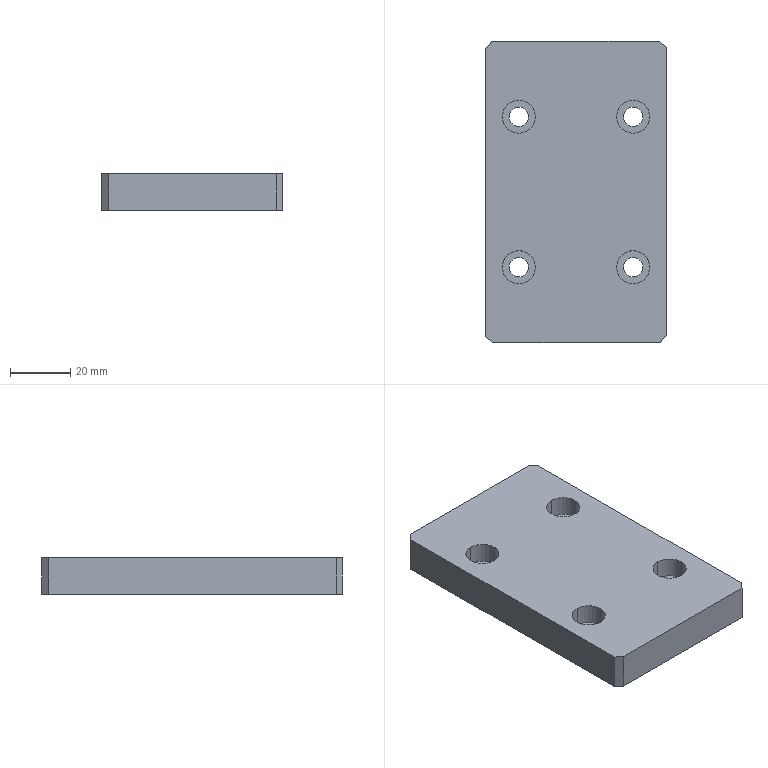Component | SolidWorks | RobotArmSupportPlate-1 | 1 solid | 30 faces | box 60 x 100 x 12 mm | volume 68632 mm3 | cylinder 16 | plane 14 | commonest cylinder face diameters 11 x8 6.4 x8
build123d program:
from build123d import *
from OCP.BRepFilletAPI import BRepFilletAPI_MakeChamfer

# Parameters (mm, degrees)
SKETCH1_W                                           = 100
SKETCH1_H                                           = 60
BOSS_EXTRUDE1_DEPTH                                 = 12
CHAMFER1_SIZE                                       = 2
CHAMFER1_SIZE2                                      = 2.384
HOLE_SIZE_ACCORDING_TO_TYPE2_OF_HEXAGON_D           = 6.4
HOLE_SIZE_ACCORDING_TO_TYPE2_OF_HEXAGON_DEPTH       = 15
HOLE_SIZE_ACCORDING_TO_TYPE2_OF_HEXAGON_CBORE_D     = 11
HOLE_SIZE_ACCORDING_TO_TYPE2_OF_HEXAGON_CBORE_DEPTH = 6.8
HOLE_SIZE_ACCORDING_TO_TYPE2_OF_HEXAGON_TIP         = 1.923


with BuildPart() as part:
    # Sketch1 → Boss-Extrude1 (new body)
    with BuildSketch(Plane.XY):
        Rectangle(SKETCH1_W, SKETCH1_H)
    extrude(amount=BOSS_EXTRUDE1_DEPTH)

    # Chamfer1: one chamfer whose edges measure the first distance from different faces: ONE call of the kernel's chamfer builder (chamfer() names one face for all edges)
    chamfer1_edges_1 = [part.edges().sort_by_distance(p)[0] for p in [
        (50, -30, 6),
    ]]
    chamfer1_side_1 = [part.faces().sort_by_distance(p)[0] for p in [
        (0, -30, 6),
    ]]
    chamfer1_edges_2 = [part.edges().sort_by_distance(p)[0] for p in [
        (-50, -30, 6),
    ]]
    chamfer1_side_2 = [part.faces().sort_by_distance(p)[0] for p in [
        (-50, 0, 6),
    ]]
    chamfer1_edges_3 = [part.edges().sort_by_distance(p)[0] for p in [
        (-50, 30, 6),
    ]]
    chamfer1_side_3 = [part.faces().sort_by_distance(p)[0] for p in [
        (0, 30, 6),
    ]]
    chamfer1_edges_4 = [part.edges().sort_by_distance(p)[0] for p in [
        (50, 30, 6),
    ]]
    chamfer1_side_4 = [part.faces().sort_by_distance(p)[0] for p in [
        (50, 0, 6),
    ]]
    chamfer1 = BRepFilletAPI_MakeChamfer(part.part.solid().wrapped)
    for e in chamfer1_edges_1:
        chamfer1.Add(CHAMFER1_SIZE, CHAMFER1_SIZE2, e.wrapped, chamfer1_side_1[0].wrapped)  # the first distance lies on this face
    for e in chamfer1_edges_2:
        chamfer1.Add(CHAMFER1_SIZE, CHAMFER1_SIZE2, e.wrapped, chamfer1_side_2[0].wrapped)  # the first distance lies on this face
    for e in chamfer1_edges_3:
        chamfer1.Add(CHAMFER1_SIZE, CHAMFER1_SIZE2, e.wrapped, chamfer1_side_3[0].wrapped)  # the first distance lies on this face
    for e in chamfer1_edges_4:
        chamfer1.Add(CHAMFER1_SIZE, CHAMFER1_SIZE2, e.wrapped, chamfer1_side_4[0].wrapped)  # the first distance lies on this face
    add(Compound.cast(chamfer1.Shape()), mode=Mode.REPLACE)

    # Hole Size_According to_Type2 of Hexagon
    with Locations(Plane.XY.offset(12)):
        with Locations((-25, 19), (-25, -19), (25, 19), (25, -19)):
            CounterBoreHole(HOLE_SIZE_ACCORDING_TO_TYPE2_OF_HEXAGON_D / 2, HOLE_SIZE_ACCORDING_TO_TYPE2_OF_HEXAGON_CBORE_D / 2, HOLE_SIZE_ACCORDING_TO_TYPE2_OF_HEXAGON_CBORE_DEPTH, depth=HOLE_SIZE_ACCORDING_TO_TYPE2_OF_HEXAGON_DEPTH)
            with Locations((0, 0, -(HOLE_SIZE_ACCORDING_TO_TYPE2_OF_HEXAGON_DEPTH + HOLE_SIZE_ACCORDING_TO_TYPE2_OF_HEXAGON_TIP / 2))):  # 118° drill point
                Cone(0, HOLE_SIZE_ACCORDING_TO_TYPE2_OF_HEXAGON_D / 2, HOLE_SIZE_ACCORDING_TO_TYPE2_OF_HEXAGON_TIP, mode=Mode.SUBTRACT)


solid = part.part

# Placed as in the assembly
solid = solid.moved(Location((-45.522, 19.945, 48.551), (0, 0, 90)))
STEP:
#1=COLOUR_RGB('',0.7922,0.8196,0.9333);
#2=FILL_AREA_STYLE_COLOUR('',#1);
#3=FILL_AREA_STYLE('',(#2));
#4=SURFACE_STYLE_FILL_AREA(#3);
#5=SURFACE_SIDE_STYLE('',(#4));
#6=SURFACE_STYLE_USAGE(.BOTH.,#5);
#7=PRESENTATION_STYLE_ASSIGNMENT((#6));
#8=CARTESIAN_POINT('',(-1.044,1.986,2.116));
#9=VERTEX_POINT('',#8);
#10=CARTESIAN_POINT('',(-1.044,1.553,2.116));
#11=VERTEX_POINT('',#10);
#12=CARTESIAN_POINT('',(-1.044,1.77,2.116));
#13=DIRECTION('',(0.,-0.,1.));
#14=DIRECTION('',(0.,-1.,0.));
#15=AXIS2_PLACEMENT_3D('',#12,#13,#14);
#16=CIRCLE('',#15,0.2165);
#17=EDGE_CURVE('',#9,#11,#16,.T.);
#18=ORIENTED_EDGE('',*,*,#17,.F.);
#19=CARTESIAN_POINT('',(-1.044,1.986,2.384));
#20=VERTEX_POINT('',#19);
#21=CARTESIAN_POINT('',(-1.044,1.986,2.384));
#22=DIRECTION('',(0.,-0.,1.));
#23=VECTOR('',#22,39.37);
#24=LINE('',#21,#23);
#25=EDGE_CURVE('',#9,#20,#24,.T.);
#26=ORIENTED_EDGE('',*,*,#25,.T.);
#27=CARTESIAN_POINT('',(-1.044,1.553,2.384));
#28=VERTEX_POINT('',#27);
#29=CARTESIAN_POINT('',(-1.044,1.77,2.384));
#30=DIRECTION('',(0.,-0.,1.));
#31=DIRECTION('',(0.,-1.,0.));
#32=AXIS2_PLACEMENT_3D('',#29,#30,#31);
#33=CIRCLE('',#32,0.2165);
#34=EDGE_CURVE('',#20,#28,#33,.T.);
#35=ORIENTED_EDGE('',*,*,#34,.T.);
#36=CARTESIAN_POINT('',(-1.044,1.553,2.384));
#37=DIRECTION('',(0.,-0.,1.));
#38=VECTOR('',#37,39.37);
#39=LINE('',#36,#38);
#40=EDGE_CURVE('',#11,#28,#39,.T.);
#41=ORIENTED_EDGE('',*,*,#40,.F.);
#42=EDGE_LOOP('',(#18,#26,#35,#41));
#43=FACE_OUTER_BOUND('',#42,.T.);
#44=CARTESIAN_POINT('',(-1.044,1.77,2.384));
#45=DIRECTION('',(0.,-0.,1.));
#46=DIRECTION('',(0.,-1.,0.));
#47=AXIS2_PLACEMENT_3D('',#44,#45,#46);
#48=CYLINDRICAL_SURFACE('',#47,0.2165);
#49=ADVANCED_FACE('',(#43),#48,.F.);
#50=CARTESIAN_POINT('',(-1.044,1.895,1.911));
#51=VERTEX_POINT('',#50);
#52=CARTESIAN_POINT('',(-1.044,1.644,1.911));
#53=VERTEX_POINT('',#52);
#54=CARTESIAN_POINT('',(-1.044,1.77,1.911));
#55=DIRECTION('',(0.,-0.,1.));
#56=DIRECTION('',(0.,-1.,0.));
#57=AXIS2_PLACEMENT_3D('',#54,#55,#56);
#58=CIRCLE('',#57,0.126);
#59=EDGE_CURVE('',#51,#53,#58,.T.);
#60=ORIENTED_EDGE('',*,*,#59,.F.);
#61=CARTESIAN_POINT('',(-1.044,1.895,2.116));
#62=VERTEX_POINT('',#61);
#63=CARTESIAN_POINT('',(-1.044,1.895,2.384));
#64=DIRECTION('',(0.,-0.,1.));
#65=VECTOR('',#64,39.37);
#66=LINE('',#63,#65);
#67=EDGE_CURVE('',#51,#62,#66,.T.);
#68=ORIENTED_EDGE('',*,*,#67,.T.);
#69=CARTESIAN_POINT('',(-1.044,1.644,2.116));
#70=VERTEX_POINT('',#69);
#71=CARTESIAN_POINT('',(-1.044,1.77,2.116));
#72=DIRECTION('',(0.,-0.,1.));
#73=DIRECTION('',(0.,-1.,0.));
#74=AXIS2_PLACEMENT_3D('',#71,#72,#73);
#75=CIRCLE('',#74,0.126);
#76=EDGE_CURVE('',#62,#70,#75,.T.);
#77=ORIENTED_EDGE('',*,*,#76,.T.);
#78=CARTESIAN_POINT('',(-1.044,1.644,2.384));
#79=DIRECTION('',(0.,-0.,1.));
#80=VECTOR('',#79,39.37);
#81=LINE('',#78,#80);
#82=EDGE_CURVE('',#53,#70,#81,.T.);
#83=ORIENTED_EDGE('',*,*,#82,.F.);
#84=EDGE_LOOP('',(#60,#68,#77,#83));
#85=FACE_OUTER_BOUND('',#84,.T.);
#86=CARTESIAN_POINT('',(-1.044,1.77,2.384));
#87=DIRECTION('',(0.,-0.,1.));
#88=DIRECTION('',(0.,-1.,0.));
#89=AXIS2_PLACEMENT_3D('',#86,#87,#88);
#90=CYLINDRICAL_SURFACE('',#89,0.126);
#91=ADVANCED_FACE('',(#85),#90,.F.);
#92=CARTESIAN_POINT('',(-2.54,1.986,2.116));
#93=VERTEX_POINT('',#92);
#94=CARTESIAN_POINT('',(-2.54,1.553,2.116));
#95=VERTEX_POINT('',#94);
#96=CARTESIAN_POINT('',(-2.54,1.77,2.116));
#97=DIRECTION('',(0.,-0.,1.));
#98=DIRECTION('',(0.,-1.,0.));
#99=AXIS2_PLACEMENT_3D('',#96,#97,#98);
#100=CIRCLE('',#99,0.2165);
#101=EDGE_CURVE('',#93,#95,#100,.T.);
#102=ORIENTED_EDGE('',*,*,#101,.F.);
#103=CARTESIAN_POINT('',(-2.54,1.986,2.384));
#104=VERTEX_POINT('',#103);
#105=CARTESIAN_POINT('',(-2.54,1.986,2.384));
#106=DIRECTION('',(0.,-0.,1.));
#107=VECTOR('',#106,39.37);
#108=LINE('',#105,#107);
#109=EDGE_CURVE('',#93,#104,#108,.T.);
#110=ORIENTED_EDGE('',*,*,#109,.T.);
#111=CARTESIAN_POINT('',(-2.54,1.553,2.384));
#112=VERTEX_POINT('',#111);
#113=CARTESIAN_POINT('',(-2.54,1.77,2.384));
#114=DIRECTION('',(0.,-0.,1.));
#115=DIRECTION('',(0.,-1.,0.));
#116=AXIS2_PLACEMENT_3D('',#113,#114,#115);
#117=CIRCLE('',#116,0.2165);
#118=EDGE_CURVE('',#104,#112,#117,.T.);
#119=ORIENTED_EDGE('',*,*,#118,.T.);
#120=CARTESIAN_POINT('',(-2.54,1.553,2.384));
#121=DIRECTION('',(0.,-0.,1.));
#122=VECTOR('',#121,39.37);
#123=LINE('',#120,#122);
#124=EDGE_CURVE('',#95,#112,#123,.T.);
#125=ORIENTED_EDGE('',*,*,#124,.F.);
#126=EDGE_LOOP('',(#102,#110,#119,#125));
#127=FACE_OUTER_BOUND('',#126,.T.);
#128=CARTESIAN_POINT('',(-2.54,1.77,2.384));
#129=DIRECTION('',(0.,-0.,1.));
#130=DIRECTION('',(0.,-1.,0.));
#131=AXIS2_PLACEMENT_3D('',#128,#129,#130);
#132=CYLINDRICAL_SURFACE('',#131,0.2165);
#133=ADVANCED_FACE('',(#127),#132,.F.);
#134=CARTESIAN_POINT('',(-2.54,1.895,1.911));
#135=VERTEX_POINT('',#134);
#136=CARTESIAN_POINT('',(-2.54,1.644,1.911));
#137=VERTEX_POINT('',#136);
#138=CARTESIAN_POINT('',(-2.54,1.77,1.911));
#139=DIRECTION('',(0.,-0.,1.));
#140=DIRECTION('',(0.,-1.,0.));
#141=AXIS2_PLACEMENT_3D('',#138,#139,#140);
#142=CIRCLE('',#141,0.126);
#143=EDGE_CURVE('',#135,#137,#142,.T.);
#144=ORIENTED_EDGE('',*,*,#143,.F.);
#145=CARTESIAN_POINT('',(-2.54,1.895,2.116));
#146=VERTEX_POINT('',#145);
#147=CARTESIAN_POINT('',(-2.54,1.895,2.384));
#148=DIRECTION('',(0.,-0.,1.));
#149=VECTOR('',#148,39.37);
#150=LINE('',#147,#149);
#151=EDGE_CURVE('',#135,#146,#150,.T.);
#152=ORIENTED_EDGE('',*,*,#151,.T.);
#153=CARTESIAN_POINT('',(-2.54,1.644,2.116));
#154=VERTEX_POINT('',#153);
#155=CARTESIAN_POINT('',(-2.54,1.77,2.116));
#156=DIRECTION('',(0.,-0.,1.));
#157=DIRECTION('',(0.,-1.,0.));
#158=AXIS2_PLACEMENT_3D('',#155,#156,#157);
#159=CIRCLE('',#158,0.126);
#160=EDGE_CURVE('',#146,#154,#159,.T.);
#161=ORIENTED_EDGE('',*,*,#160,.T.);
#162=CARTESIAN_POINT('',(-2.54,1.644,2.384));
#163=DIRECTION('',(0.,-0.,1.));
#164=VECTOR('',#163,39.37);
#165=LINE('',#162,#164);
#166=EDGE_CURVE('',#137,#154,#165,.T.);
#167=ORIENTED_EDGE('',*,*,#166,.F.);
#168=EDGE_LOOP('',(#144,#152,#161,#167));
#169=FACE_OUTER_BOUND('',#168,.T.);
#170=CARTESIAN_POINT('',(-2.54,1.77,2.384));
#171=DIRECTION('',(0.,-0.,1.));
#172=DIRECTION('',(0.,-1.,0.));
#173=AXIS2_PLACEMENT_3D('',#170,#171,#172);
#174=CYLINDRICAL_SURFACE('',#173,0.126);
#175=ADVANCED_FACE('',(#169),#174,.F.);
#176=CARTESIAN_POINT('',(-1.044,0.01754,2.116));
#177=VERTEX_POINT('',#176);
#178=CARTESIAN_POINT('',(-1.044,-0.4155,2.116));
#179=VERTEX_POINT('',#178);
#180=CARTESIAN_POINT('',(-1.044,-0.199,2.116));
#181=DIRECTION('',(0.,-0.,1.));
#182=DIRECTION('',(0.,-1.,0.));
#183=AXIS2_PLACEMENT_3D('',#180,#181,#182);
#184=CIRCLE('',#183,0.2165);
#185=EDGE_CURVE('',#177,#179,#184,.T.);
#186=ORIENTED_EDGE('',*,*,#185,.F.);
#187=CARTESIAN_POINT('',(-1.044,0.01754,2.384));
#188=VERTEX_POINT('',#187);
#189=CARTESIAN_POINT('',(-1.044,0.01754,2.384));
#190=DIRECTION('',(0.,-0.,1.));
#191=VECTOR('',#190,39.37);
#192=LINE('',#189,#191);
#193=EDGE_CURVE('',#177,#188,#192,.T.);
#194=ORIENTED_EDGE('',*,*,#193,.T.);
#195=CARTESIAN_POINT('',(-1.044,-0.4155,2.384));
#196=VERTEX_POINT('',#195);
#197=CARTESIAN_POINT('',(-1.044,-0.199,2.384));
#198=DIRECTION('',(0.,-0.,1.));
#199=DIRECTION('',(0.,-1.,0.));
#200=AXIS2_PLACEMENT_3D('',#197,#198,#199);
#201=CIRCLE('',#200,0.2165);
#202=EDGE_CURVE('',#188,#196,#201,.T.);
#203=ORIENTED_EDGE('',*,*,#202,.T.);
#204=CARTESIAN_POINT('',(-1.044,-0.4155,2.384));
#205=DIRECTION('',(0.,-0.,1.));
#206=VECTOR('',#205,39.37);
#207=LINE('',#204,#206);
#208=EDGE_CURVE('',#179,#196,#207,.T.);
#209=ORIENTED_EDGE('',*,*,#208,.F.);
#210=EDGE_LOOP('',(#186,#194,#203,#209));
#211=FACE_OUTER_BOUND('',#210,.T.);
#212=CARTESIAN_POINT('',(-1.044,-0.199,2.384));
#213=DIRECTION('',(0.,-0.,1.));
#214=DIRECTION('',(0.,-1.,0.));
#215=AXIS2_PLACEMENT_3D('',#212,#213,#214);
#216=CYLINDRICAL_SURFACE('',#215,0.2165);
#217=ADVANCED_FACE('',(#211),#216,.F.);
#218=CARTESIAN_POINT('',(-1.044,-0.07302,1.911));
#219=VERTEX_POINT('',#218);
#220=CARTESIAN_POINT('',(-1.044,-0.325,1.911));
#221=VERTEX_POINT('',#220);
#222=CARTESIAN_POINT('',(-1.044,-0.199,1.911));
#223=DIRECTION('',(0.,-0.,1.));
#224=DIRECTION('',(0.,-1.,0.));
#225=AXIS2_PLACEMENT_3D('',#222,#223,#224);
#226=CIRCLE('',#225,0.126);
#227=EDGE_CURVE('',#219,#221,#226,.T.);
#228=ORIENTED_EDGE('',*,*,#227,.F.);
#229=CARTESIAN_POINT('',(-1.044,-0.07302,2.116));
#230=VERTEX_POINT('',#229);
#231=CARTESIAN_POINT('',(-1.044,-0.07302,2.384));
#232=DIRECTION('',(0.,-0.,1.));
#233=VECTOR('',#232,39.37);
#234=LINE('',#231,#233);
#235=EDGE_CURVE('',#219,#230,#234,.T.);
#236=ORIENTED_EDGE('',*,*,#235,.T.);
#237=CARTESIAN_POINT('',(-1.044,-0.325,2.116));
#238=VERTEX_POINT('',#237);
#239=CARTESIAN_POINT('',(-1.044,-0.199,2.116));
#240=DIRECTION('',(0.,-0.,1.));
#241=DIRECTION('',(0.,-1.,0.));
#242=AXIS2_PLACEMENT_3D('',#239,#240,#241);
#243=CIRCLE('',#242,0.126);
#244=EDGE_CURVE('',#230,#238,#243,.T.);
#245=ORIENTED_EDGE('',*,*,#244,.T.);
#246=CARTESIAN_POINT('',(-1.044,-0.325,2.384));
#247=DIRECTION('',(0.,-0.,1.));
#248=VECTOR('',#247,39.37);
#249=LINE('',#246,#248);
#250=EDGE_CURVE('',#221,#238,#249,.T.);
#251=ORIENTED_EDGE('',*,*,#250,.F.);
#252=EDGE_LOOP('',(#228,#236,#245,#251));
#253=FACE_OUTER_BOUND('',#252,.T.);
#254=CARTESIAN_POINT('',(-1.044,-0.199,2.384));
#255=DIRECTION('',(0.,-0.,1.));
#256=DIRECTION('',(0.,-1.,0.));
#257=AXIS2_PLACEMENT_3D('',#254,#255,#256);
#258=CYLINDRICAL_SURFACE('',#257,0.126);
#259=ADVANCED_FACE('',(#253),#258,.F.);
#260=CARTESIAN_POINT('',(-2.54,0.01754,2.116));
#261=VERTEX_POINT('',#260);
#262=CARTESIAN_POINT('',(-2.54,-0.4155,2.116));
#263=VERTEX_POINT('',#262);
#264=CARTESIAN_POINT('',(-2.54,-0.199,2.116));
#265=DIRECTION('',(0.,-0.,1.));
#266=DIRECTION('',(0.,-1.,0.));
#267=AXIS2_PLACEMENT_3D('',#264,#265,#266);
#268=CIRCLE('',#267,0.2165);
#269=EDGE_CURVE('',#261,#263,#268,.T.);
#270=ORIENTED_EDGE('',*,*,#269,.F.);
#271=CARTESIAN_POINT('',(-2.54,0.01754,2.384));
#272=VERTEX_POINT('',#271);
#273=CARTESIAN_POINT('',(-2.54,0.01754,2.384));
#274=DIRECTION('',(0.,-0.,1.));
#275=VECTOR('',#274,39.37);
#276=LINE('',#273,#275);
#277=EDGE_CURVE('',#261,#272,#276,.T.);
#278=ORIENTED_EDGE('',*,*,#277,.T.);
#279=CARTESIAN_POINT('',(-2.54,-0.4155,2.384));
#280=VERTEX_POINT('',#279);
#281=CARTESIAN_POINT('',(-2.54,-0.199,2.384));
#282=DIRECTION('',(0.,-0.,1.));
#283=DIRECTION('',(0.,-1.,0.));
#284=AXIS2_PLACEMENT_3D('',#281,#282,#283);
#285=CIRCLE('',#284,0.2165);
#286=EDGE_CURVE('',#272,#280,#285,.T.);
#287=ORIENTED_EDGE('',*,*,#286,.T.);
#288=CARTESIAN_POINT('',(-2.54,-0.4155,2.384));
#289=DIRECTION('',(0.,-0.,1.));
#290=VECTOR('',#289,39.37);
#291=LINE('',#288,#290);
#292=EDGE_CURVE('',#263,#280,#291,.T.);
#293=ORIENTED_EDGE('',*,*,#292,.F.);
#294=EDGE_LOOP('',(#270,#278,#287,#293));
#295=FACE_OUTER_BOUND('',#294,.T.);
#296=CARTESIAN_POINT('',(-2.54,-0.199,2.384));
#297=DIRECTION('',(0.,-0.,1.));
#298=DIRECTION('',(0.,-1.,0.));
#299=AXIS2_PLACEMENT_3D('',#296,#297,#298);
#300=CYLINDRICAL_SURFACE('',#299,0.2165);
#301=ADVANCED_FACE('',(#295),#300,.F.);
#302=CARTESIAN_POINT('',(-2.54,-0.07302,1.911));
#303=VERTEX_POINT('',#302);
#304=CARTESIAN_POINT('',(-2.54,-0.325,1.911));
#305=VERTEX_POINT('',#304);
#306=CARTESIAN_POINT('',(-2.54,-0.199,1.911));
#307=DIRECTION('',(0.,-0.,1.));
#308=DIRECTION('',(0.,-1.,0.));
#309=AXIS2_PLACEMENT_3D('',#306,#307,#308);
#310=CIRCLE('',#309,0.126);
#311=EDGE_CURVE('',#303,#305,#310,.T.);
#312=ORIENTED_EDGE('',*,*,#311,.F.);
#313=CARTESIAN_POINT('',(-2.54,-0.07302,2.116));
#314=VERTEX_POINT('',#313);
#315=CARTESIAN_POINT('',(-2.54,-0.07302,2.384));
#316=DIRECTION('',(0.,-0.,1.));
#317=VECTOR('',#316,39.37);
#318=LINE('',#315,#317);
#319=EDGE_CURVE('',#303,#314,#318,.T.);
#320=ORIENTED_EDGE('',*,*,#319,.T.);
#321=CARTESIAN_POINT('',(-2.54,-0.325,2.116));
#322=VERTEX_POINT('',#321);
#323=CARTESIAN_POINT('',(-2.54,-0.199,2.116));
#324=DIRECTION('',(0.,-0.,1.));
#325=DIRECTION('',(0.,-1.,0.));
#326=AXIS2_PLACEMENT_3D('',#323,#324,#325);
#327=CIRCLE('',#326,0.126);
#328=EDGE_CURVE('',#314,#322,#327,.T.);
#329=ORIENTED_EDGE('',*,*,#328,.T.);
#330=CARTESIAN_POINT('',(-2.54,-0.325,2.384));
#331=DIRECTION('',(0.,-0.,1.));
#332=VECTOR('',#331,39.37);
#333=LINE('',#330,#332);
#334=EDGE_CURVE('',#305,#322,#333,.T.);
#335=ORIENTED_EDGE('',*,*,#334,.F.);
#336=EDGE_LOOP('',(#312,#320,#329,#335));
#337=FACE_OUTER_BOUND('',#336,.T.);
#338=CARTESIAN_POINT('',(-2.54,-0.199,2.384));
#339=DIRECTION('',(0.,-0.,1.));
#340=DIRECTION('',(0.,-1.,0.));
#341=AXIS2_PLACEMENT_3D('',#338,#339,#340);
#342=CYLINDRICAL_SURFACE('',#341,0.126);
#343=ADVANCED_FACE('',(#337),#342,.F.);
#344=CARTESIAN_POINT('',(-2.879,-1.183,2.384));
#345=VERTEX_POINT('',#344);
#346=CARTESIAN_POINT('',(-0.6899,-1.183,2.384));
#347=VERTEX_POINT('',#346);
#348=CARTESIAN_POINT('',(-0.6111,-1.183,2.384));
#349=DIRECTION('',(1.,0.,-0.));
#350=VECTOR('',#349,39.37);
#351=LINE('',#348,#350);
#352=EDGE_CURVE('',#345,#347,#351,.T.);
#353=ORIENTED_EDGE('',*,*,#352,.F.);
#354=CARTESIAN_POINT('',(-2.879,-1.183,1.911));
#355=VERTEX_POINT('',#354);
#356=CARTESIAN_POINT('',(-2.879,-1.183,2.384));
#357=DIRECTION('',(-0.,0.,-1.));
#358=VECTOR('',#357,39.37);
#359=LINE('',#356,#358);
#360=EDGE_CURVE('',#345,#355,#359,.T.);
#361=ORIENTED_EDGE('',*,*,#360,.T.);
#362=CARTESIAN_POINT('',(-0.6899,-1.183,1.911));
#363=VERTEX_POINT('',#362);
#364=CARTESIAN_POINT('',(-0.6111,-1.183,1.911));
#365=DIRECTION('',(1.,0.,-0.));
#366=VECTOR('',#365,39.37);
#367=LINE('',#364,#366);
#368=EDGE_CURVE('',#355,#363,#367,.T.);
#369=ORIENTED_EDGE('',*,*,#368,.T.);
#370=CARTESIAN_POINT('',(-0.6899,-1.183,2.384));
#371=DIRECTION('',(0.,-0.,1.));
#372=VECTOR('',#371,39.37);
#373=LINE('',#370,#372);
#374=EDGE_CURVE('',#363,#347,#373,.T.);
#375=ORIENTED_EDGE('',*,*,#374,.T.);
#376=EDGE_LOOP('',(#353,#361,#369,#375));
#377=FACE_OUTER_BOUND('',#376,.T.);
#378=CARTESIAN_POINT('',(-0.6111,-1.183,2.384));
#379=DIRECTION('',(-0.,1.,0.));
#380=DIRECTION('',(-1.,-0.,0.));
#381=AXIS2_PLACEMENT_3D('',#378,#379,#380);
#382=PLANE('',#381);
#383=ADVANCED_FACE('',(#377),#382,.F.);
#384=CARTESIAN_POINT('',(-0.6111,-1.089,1.911));
#385=VERTEX_POINT('',#384);
#386=CARTESIAN_POINT('',(-0.6111,2.675,1.911));
#387=VERTEX_POINT('',#386);
#388=CARTESIAN_POINT('',(-0.6111,2.754,1.911));
#389=DIRECTION('',(-0.,1.,0.));
#390=VECTOR('',#389,39.37);
#391=LINE('',#388,#390);
#392=EDGE_CURVE('',#385,#387,#391,.T.);
#393=ORIENTED_EDGE('',*,*,#392,.T.);
#394=CARTESIAN_POINT('',(-0.6111,2.675,2.384));
#395=VERTEX_POINT('',#394);
#396=CARTESIAN_POINT('',(-0.6111,2.675,2.384));
#397=DIRECTION('',(0.,-0.,1.));
#398=VECTOR('',#397,39.37);
#399=LINE('',#396,#398);
#400=EDGE_CURVE('',#387,#395,#399,.T.);
#401=ORIENTED_EDGE('',*,*,#400,.T.);
#402=CARTESIAN_POINT('',(-0.6111,-1.089,2.384));
#403=VERTEX_POINT('',#402);
#404=CARTESIAN_POINT('',(-0.6111,2.754,2.384));
#405=DIRECTION('',(-0.,1.,0.));
#406=VECTOR('',#405,39.37);
#407=LINE('',#404,#406);
#408=EDGE_CURVE('',#403,#395,#407,.T.);
#409=ORIENTED_EDGE('',*,*,#408,.F.);
#410=CARTESIAN_POINT('',(-0.6111,-1.089,2.384));
#411=DIRECTION('',(-0.,0.,-1.));
#412=VECTOR('',#411,39.37);
#413=LINE('',#410,#412);
#414=EDGE_CURVE('',#403,#385,#413,.T.);
#415=ORIENTED_EDGE('',*,*,#414,.T.);
#416=EDGE_LOOP('',(#393,#401,#409,#415));
#417=FACE_OUTER_BOUND('',#416,.T.);
#418=CARTESIAN_POINT('',(-0.6111,2.754,2.384));
#419=DIRECTION('',(-1.,-0.,0.));
#420=DIRECTION('',(-0.,0.,-1.));
#421=AXIS2_PLACEMENT_3D('',#418,#419,#420);
#422=PLANE('',#421);
#423=ADVANCED_FACE('',(#417),#422,.F.);
#424=CARTESIAN_POINT('',(-0.705,2.754,1.911));
#425=VERTEX_POINT('',#424);
#426=CARTESIAN_POINT('',(-2.895,2.754,1.911));
#427=VERTEX_POINT('',#426);
#428=CARTESIAN_POINT('',(-0.6111,2.754,1.911));
#429=DIRECTION('',(-1.,-0.,0.));
#430=VECTOR('',#429,39.37);
#431=LINE('',#428,#430);
#432=EDGE_CURVE('',#425,#427,#431,.T.);
#433=ORIENTED_EDGE('',*,*,#432,.T.);
#434=CARTESIAN_POINT('',(-2.895,2.754,2.384));
#435=VERTEX_POINT('',#434);
#436=CARTESIAN_POINT('',(-2.895,2.754,2.384));
#437=DIRECTION('',(0.,-0.,1.));
#438=VECTOR('',#437,39.37);
#439=LINE('',#436,#438);
#440=EDGE_CURVE('',#427,#435,#439,.T.);
#441=ORIENTED_EDGE('',*,*,#440,.T.);
#442=CARTESIAN_POINT('',(-0.705,2.754,2.384));
#443=VERTEX_POINT('',#442);
#444=CARTESIAN_POINT('',(-0.6111,2.754,2.384));
#445=DIRECTION('',(-1.,-0.,0.));
#446=VECTOR('',#445,39.37);
#447=LINE('',#444,#446);
#448=EDGE_CURVE('',#443,#435,#447,.T.);
#449=ORIENTED_EDGE('',*,*,#448,.F.);
#450=CARTESIAN_POINT('',(-0.705,2.754,2.384));
#451=DIRECTION('',(-0.,0.,-1.));
#452=VECTOR('',#451,39.37);
#453=LINE('',#450,#452);
#454=EDGE_CURVE('',#443,#425,#453,.T.);
#455=ORIENTED_EDGE('',*,*,#454,.T.);
#456=EDGE_LOOP('',(#433,#441,#449,#455));
#457=FACE_OUTER_BOUND('',#456,.T.);
#458=CARTESIAN_POINT('',(-0.6111,2.754,2.384));
#459=DIRECTION('',(0.,-1.,-0.));
#460=DIRECTION('',(-0.,0.,-1.));
#461=AXIS2_PLACEMENT_3D('',#458,#459,#460);
#462=PLANE('',#461);
#463=ADVANCED_FACE('',(#457),#462,.F.);
#464=CARTESIAN_POINT('',(-2.973,2.66,1.911));
#465=VERTEX_POINT('',#464);
#466=CARTESIAN_POINT('',(-2.973,-1.105,1.911));
#467=VERTEX_POINT('',#466);
#468=CARTESIAN_POINT('',(-2.973,2.754,1.911));
#469=DIRECTION('',(0.,-1.,-0.));
#470=VECTOR('',#469,39.37);
#471=LINE('',#468,#470);
#472=EDGE_CURVE('',#465,#467,#471,.T.);
#473=ORIENTED_EDGE('',*,*,#472,.T.);
#474=CARTESIAN_POINT('',(-2.973,-1.105,2.384));
#475=VERTEX_POINT('',#474);
#476=CARTESIAN_POINT('',(-2.973,-1.105,2.384));
#477=DIRECTION('',(0.,-0.,1.));
#478=VECTOR('',#477,39.37);
#479=LINE('',#476,#478);
#480=EDGE_CURVE('',#467,#475,#479,.T.);
#481=ORIENTED_EDGE('',*,*,#480,.T.);
#482=CARTESIAN_POINT('',(-2.973,2.66,2.384));
#483=VERTEX_POINT('',#482);
#484=CARTESIAN_POINT('',(-2.973,2.754,2.384));
#485=DIRECTION('',(0.,-1.,-0.));
#486=VECTOR('',#485,39.37);
#487=LINE('',#484,#486);
#488=EDGE_CURVE('',#483,#475,#487,.T.);
#489=ORIENTED_EDGE('',*,*,#488,.F.);
#490=CARTESIAN_POINT('',(-2.973,2.66,2.384));
#491=DIRECTION('',(-0.,0.,-1.));
#492=VECTOR('',#491,39.37);
#493=LINE('',#490,#492);
#494=EDGE_CURVE('',#483,#465,#493,.T.);
#495=ORIENTED_EDGE('',*,*,#494,.T.);
#496=EDGE_LOOP('',(#473,#481,#489,#495));
#497=FACE_OUTER_BOUND('',#496,.T.);
#498=CARTESIAN_POINT('',(-2.973,2.754,2.384));
#499=DIRECTION('',(1.,0.,-0.));
#500=DIRECTION('',(0.,-0.,1.));
#501=AXIS2_PLACEMENT_3D('',#498,#499,#500);
#502=PLANE('',#501);
#503=ADVANCED_FACE('',(#497),#502,.F.);
#504=CARTESIAN_POINT('',(-1.044,1.77,2.384));
#505=DIRECTION('',(0.,-0.,1.));
#506=DIRECTION('',(0.,-1.,0.));
#507=AXIS2_PLACEMENT_3D('',#504,#505,#506);
#508=CIRCLE('',#507,0.2165);
#509=EDGE_CURVE('',#28,#20,#508,.T.);
#510=ORIENTED_EDGE('',*,*,#509,.F.);
#511=ORIENTED_EDGE('',*,*,#34,.F.);
#512=EDGE_LOOP('',(#510,#511));
#513=FACE_BOUND('',#512,.T.);
#514=CARTESIAN_POINT('',(-2.54,1.77,2.384));
#515=DIRECTION('',(0.,-0.,1.));
#516=DIRECTION('',(0.,-1.,0.));
#517=AXIS2_PLACEMENT_3D('',#514,#515,#516);
#518=CIRCLE('',#517,0.2165);
#519=EDGE_CURVE('',#112,#104,#518,.T.);
#520=ORIENTED_EDGE('',*,*,#519,.F.);
#521=ORIENTED_EDGE('',*,*,#118,.F.);
#522=EDGE_LOOP('',(#520,#521));
#523=FACE_BOUND('',#522,.T.);
#524=CARTESIAN_POINT('',(-1.044,-0.199,2.384));
#525=DIRECTION('',(0.,-0.,1.));
#526=DIRECTION('',(0.,-1.,0.));
#527=AXIS2_PLACEMENT_3D('',#524,#525,#526);
#528=CIRCLE('',#527,0.2165);
#529=EDGE_CURVE('',#196,#188,#528,.T.);
#530=ORIENTED_EDGE('',*,*,#529,.F.);
#531=ORIENTED_EDGE('',*,*,#202,.F.);
#532=EDGE_LOOP('',(#530,#531));
#533=FACE_BOUND('',#532,.T.);
#534=CARTESIAN_POINT('',(-2.54,-0.199,2.384));
#535=DIRECTION('',(0.,-0.,1.));
#536=DIRECTION('',(0.,-1.,0.));
#537=AXIS2_PLACEMENT_3D('',#534,#535,#536);
#538=CIRCLE('',#537,0.2165);
#539=EDGE_CURVE('',#280,#272,#538,.T.);
#540=ORIENTED_EDGE('',*,*,#539,.F.);
#541=ORIENTED_EDGE('',*,*,#286,.F.);
#542=EDGE_LOOP('',(#540,#541));
#543=FACE_BOUND('',#542,.T.);
#544=ORIENTED_EDGE('',*,*,#488,.T.);
#545=CARTESIAN_POINT('',(-3.211,-0.9053,2.384));
#546=DIRECTION('',(0.766,-0.6428,-0.));
#547=VECTOR('',#546,39.37);
#548=LINE('',#545,#547);
#549=EDGE_CURVE('',#475,#345,#548,.T.);
#550=ORIENTED_EDGE('',*,*,#549,.T.);
#551=ORIENTED_EDGE('',*,*,#352,.T.);
#552=CARTESIAN_POINT('',(-0.176,-0.5709,2.384));
#553=DIRECTION('',(0.6428,0.766,0.));
#554=VECTOR('',#553,39.37);
#555=LINE('',#552,#554);
#556=EDGE_CURVE('',#347,#403,#555,.T.);
#557=ORIENTED_EDGE('',*,*,#556,.T.);
#558=ORIENTED_EDGE('',*,*,#408,.T.);
#559=CARTESIAN_POINT('',(-0.3737,2.476,2.384));
#560=DIRECTION('',(-0.766,0.6428,0.));
#561=VECTOR('',#560,39.37);
#562=LINE('',#559,#561);
#563=EDGE_CURVE('',#395,#443,#562,.T.);
#564=ORIENTED_EDGE('',*,*,#563,.T.);
#565=ORIENTED_EDGE('',*,*,#448,.T.);
#566=CARTESIAN_POINT('',(-3.408,2.141,2.384));
#567=DIRECTION('',(-0.6428,-0.766,-0.));
#568=VECTOR('',#567,39.37);
#569=LINE('',#566,#568);
#570=EDGE_CURVE('',#435,#483,#569,.T.);
#571=ORIENTED_EDGE('',*,*,#570,.T.);
#572=EDGE_LOOP('',(#544,#550,#551,#557,#558,#564,#565,#571));
#573=FACE_OUTER_BOUND('',#572,.T.);
#574=CARTESIAN_POINT('',(-1.792,0.7853,2.384));
#575=DIRECTION('',(0.,-0.,1.));
#576=DIRECTION('',(0.,-1.,-0.));
#577=AXIS2_PLACEMENT_3D('',#574,#575,#576);
#578=PLANE('',#577);
#579=ADVANCED_FACE('',(#513,#523,#533,#543,#573),#578,.T.);
#580=CARTESIAN_POINT('',(-1.044,1.77,1.911));
#581=DIRECTION('',(0.,-0.,1.));
#582=DIRECTION('',(0.,-1.,0.));
#583=AXIS2_PLACEMENT_3D('',#580,#581,#582);
#584=CIRCLE('',#583,0.126);
#585=EDGE_CURVE('',#53,#51,#584,.T.);
#586=ORIENTED_EDGE('',*,*,#585,.T.);
#587=ORIENTED_EDGE('',*,*,#59,.T.);
#588=EDGE_LOOP('',(#586,#587));
#589=FACE_BOUND('',#588,.T.);
#590=CARTESIAN_POINT('',(-2.54,1.77,1.911));
#591=DIRECTION('',(0.,-0.,1.));
#592=DIRECTION('',(0.,-1.,0.));
#593=AXIS2_PLACEMENT_3D('',#590,#591,#592);
#594=CIRCLE('',#593,0.126);
#595=EDGE_CURVE('',#137,#135,#594,.T.);
#596=ORIENTED_EDGE('',*,*,#595,.T.);
#597=ORIENTED_EDGE('',*,*,#143,.T.);
#598=EDGE_LOOP('',(#596,#597));
#599=FACE_BOUND('',#598,.T.);
#600=CARTESIAN_POINT('',(-1.044,-0.199,1.911));
#601=DIRECTION('',(0.,-0.,1.));
#602=DIRECTION('',(0.,-1.,0.));
#603=AXIS2_PLACEMENT_3D('',#600,#601,#602);
#604=CIRCLE('',#603,0.126);
#605=EDGE_CURVE('',#221,#219,#604,.T.);
#606=ORIENTED_EDGE('',*,*,#605,.T.);
#607=ORIENTED_EDGE('',*,*,#227,.T.);
#608=EDGE_LOOP('',(#606,#607));
#609=FACE_BOUND('',#608,.T.);
#610=CARTESIAN_POINT('',(-2.54,-0.199,1.911));
#611=DIRECTION('',(0.,-0.,1.));
#612=DIRECTION('',(0.,-1.,0.));
#613=AXIS2_PLACEMENT_3D('',#610,#611,#612);
#614=CIRCLE('',#613,0.126);
#615=EDGE_CURVE('',#305,#303,#614,.T.);
#616=ORIENTED_EDGE('',*,*,#615,.T.);
#617=ORIENTED_EDGE('',*,*,#311,.T.);
#618=EDGE_LOOP('',(#616,#617));
#619=FACE_BOUND('',#618,.T.);
#620=ORIENTED_EDGE('',*,*,#368,.F.);
#621=CARTESIAN_POINT('',(-2.879,-1.183,1.911));
#622=DIRECTION('',(-0.766,0.6428,0.));
#623=VECTOR('',#622,39.37);
#624=LINE('',#621,#623);
#625=EDGE_CURVE('',#355,#467,#624,.T.);
#626=ORIENTED_EDGE('',*,*,#625,.T.);
#627=ORIENTED_EDGE('',*,*,#472,.F.);
#628=CARTESIAN_POINT('',(-2.973,2.66,1.911));
#629=DIRECTION('',(0.6428,0.766,0.));
#630=VECTOR('',#629,39.37);
#631=LINE('',#628,#630);
#632=EDGE_CURVE('',#465,#427,#631,.T.);
#633=ORIENTED_EDGE('',*,*,#632,.T.);
#634=ORIENTED_EDGE('',*,*,#432,.F.);
#635=CARTESIAN_POINT('',(-0.705,2.754,1.911));
#636=DIRECTION('',(0.766,-0.6428,-0.));
#637=VECTOR('',#636,39.37);
#638=LINE('',#635,#637);
#639=EDGE_CURVE('',#425,#387,#638,.T.);
#640=ORIENTED_EDGE('',*,*,#639,.T.);
#641=ORIENTED_EDGE('',*,*,#392,.F.);
#642=CARTESIAN_POINT('',(-0.6111,-1.089,1.911));
#643=DIRECTION('',(-0.6428,-0.766,-0.));
#644=VECTOR('',#643,39.37);
#645=LINE('',#642,#644);
#646=EDGE_CURVE('',#385,#363,#645,.T.);
#647=ORIENTED_EDGE('',*,*,#646,.T.);
#648=EDGE_LOOP('',(#620,#626,#627,#633,#634,#640,#641,#647));
#649=FACE_OUTER_BOUND('',#648,.T.);
#650=CARTESIAN_POINT('',(-1.792,0.7853,1.911));
#651=DIRECTION('',(0.,-0.,1.));
#652=DIRECTION('',(0.,-1.,-0.));
#653=AXIS2_PLACEMENT_3D('',#650,#651,#652);
#654=PLANE('',#653);
#655=ADVANCED_FACE('',(#589,#599,#609,#619,#649),#654,.F.);
#656=ORIENTED_EDGE('',*,*,#549,.F.);
#657=ORIENTED_EDGE('',*,*,#480,.F.);
#658=ORIENTED_EDGE('',*,*,#625,.F.);
#659=ORIENTED_EDGE('',*,*,#360,.F.);
#660=EDGE_LOOP('',(#656,#657,#658,#659));
#661=FACE_OUTER_BOUND('',#660,.T.);
#662=CARTESIAN_POINT('',(-2.879,-1.183,2.384));
#663=DIRECTION('',(0.6428,0.766,0.));
#664=DIRECTION('',(-0.,0.,-1.));
#665=AXIS2_PLACEMENT_3D('',#662,#663,#664);
#666=PLANE('',#665);
#667=ADVANCED_FACE('',(#661),#666,.F.);
#668=ORIENTED_EDGE('',*,*,#570,.F.);
#669=ORIENTED_EDGE('',*,*,#440,.F.);
#670=ORIENTED_EDGE('',*,*,#632,.F.);
#671=ORIENTED_EDGE('',*,*,#494,.F.);
#672=EDGE_LOOP('',(#668,#669,#670,#671));
#673=FACE_OUTER_BOUND('',#672,.T.);
#674=CARTESIAN_POINT('',(-2.973,2.66,2.384));
#675=DIRECTION('',(0.766,-0.6428,-0.));
#676=DIRECTION('',(-0.,0.,-1.));
#677=AXIS2_PLACEMENT_3D('',#674,#675,#676);
#678=PLANE('',#677);
#679=ADVANCED_FACE('',(#673),#678,.F.);
#680=ORIENTED_EDGE('',*,*,#563,.F.);
#681=ORIENTED_EDGE('',*,*,#400,.F.);
#682=ORIENTED_EDGE('',*,*,#639,.F.);
#683=ORIENTED_EDGE('',*,*,#454,.F.);
#684=EDGE_LOOP('',(#680,#681,#682,#683));
#685=FACE_OUTER_BOUND('',#684,.T.);
#686=CARTESIAN_POINT('',(-0.705,2.754,2.384));
#687=DIRECTION('',(-0.6428,-0.766,-0.));
#688=DIRECTION('',(-0.,0.,-1.));
#689=AXIS2_PLACEMENT_3D('',#686,#687,#688);
#690=PLANE('',#689);
#691=ADVANCED_FACE('',(#685),#690,.F.);
#692=ORIENTED_EDGE('',*,*,#556,.F.);
#693=ORIENTED_EDGE('',*,*,#374,.F.);
#694=ORIENTED_EDGE('',*,*,#646,.F.);
#695=ORIENTED_EDGE('',*,*,#414,.F.);
#696=EDGE_LOOP('',(#692,#693,#694,#695));
#697=FACE_OUTER_BOUND('',#696,.T.);
#698=CARTESIAN_POINT('',(-0.6111,-1.089,2.384));
#699=DIRECTION('',(-0.766,0.6428,0.));
#700=DIRECTION('',(-0.,0.,-1.));
#701=AXIS2_PLACEMENT_3D('',#698,#699,#700);
#702=PLANE('',#701);
#703=ADVANCED_FACE('',(#697),#702,.F.);
#704=ORIENTED_EDGE('',*,*,#319,.F.);
#705=ORIENTED_EDGE('',*,*,#615,.F.);
#706=ORIENTED_EDGE('',*,*,#334,.T.);
#707=CARTESIAN_POINT('',(-2.54,-0.199,2.116));
#708=DIRECTION('',(0.,-0.,1.));
#709=DIRECTION('',(0.,-1.,0.));
#710=AXIS2_PLACEMENT_3D('',#707,#708,#709);
#711=CIRCLE('',#710,0.126);
#712=EDGE_CURVE('',#322,#314,#711,.T.);
#713=ORIENTED_EDGE('',*,*,#712,.T.);
#714=EDGE_LOOP('',(#704,#705,#706,#713));
#715=FACE_OUTER_BOUND('',#714,.T.);
#716=CARTESIAN_POINT('',(-2.54,-0.199,2.384));
#717=DIRECTION('',(0.,-0.,1.));
#718=DIRECTION('',(0.,-1.,0.));
#719=AXIS2_PLACEMENT_3D('',#716,#717,#718);
#720=CYLINDRICAL_SURFACE('',#719,0.126);
#721=ADVANCED_FACE('',(#715),#720,.F.);
#722=ORIENTED_EDGE('',*,*,#712,.F.);
#723=ORIENTED_EDGE('',*,*,#328,.F.);
#724=EDGE_LOOP('',(#722,#723));
#725=FACE_BOUND('',#724,.T.);
#726=CARTESIAN_POINT('',(-2.54,-0.199,2.116));
#727=DIRECTION('',(0.,-0.,1.));
#728=DIRECTION('',(0.,-1.,0.));
#729=AXIS2_PLACEMENT_3D('',#726,#727,#728);
#730=CIRCLE('',#729,0.2165);
#731=EDGE_CURVE('',#263,#261,#730,.T.);
#732=ORIENTED_EDGE('',*,*,#731,.T.);
#733=ORIENTED_EDGE('',*,*,#269,.T.);
#734=EDGE_LOOP('',(#732,#733));
#735=FACE_OUTER_BOUND('',#734,.T.);
#736=CARTESIAN_POINT('',(-2.54,-0.325,2.116));
#737=DIRECTION('',(-0.,0.,-1.));
#738=DIRECTION('',(-0.,1.,0.));
#739=AXIS2_PLACEMENT_3D('',#736,#737,#738);
#740=PLANE('',#739);
#741=ADVANCED_FACE('',(#725,#735),#740,.F.);
#742=ORIENTED_EDGE('',*,*,#277,.F.);
#743=ORIENTED_EDGE('',*,*,#731,.F.);
#744=ORIENTED_EDGE('',*,*,#292,.T.);
#745=ORIENTED_EDGE('',*,*,#539,.T.);
#746=EDGE_LOOP('',(#742,#743,#744,#745));
#747=FACE_OUTER_BOUND('',#746,.T.);
#748=CARTESIAN_POINT('',(-2.54,-0.199,2.384));
#749=DIRECTION('',(0.,-0.,1.));
#750=DIRECTION('',(0.,-1.,0.));
#751=AXIS2_PLACEMENT_3D('',#748,#749,#750);
#752=CYLINDRICAL_SURFACE('',#751,0.2165);
#753=ADVANCED_FACE('',(#747),#752,.F.);
#754=ORIENTED_EDGE('',*,*,#235,.F.);
#755=ORIENTED_EDGE('',*,*,#605,.F.);
#756=ORIENTED_EDGE('',*,*,#250,.T.);
#757=CARTESIAN_POINT('',(-1.044,-0.199,2.116));
#758=DIRECTION('',(0.,-0.,1.));
#759=DIRECTION('',(0.,-1.,0.));
#760=AXIS2_PLACEMENT_3D('',#757,#758,#759);
#761=CIRCLE('',#760,0.126);
#762=EDGE_CURVE('',#238,#230,#761,.T.);
#763=ORIENTED_EDGE('',*,*,#762,.T.);
#764=EDGE_LOOP('',(#754,#755,#756,#763));
#765=FACE_OUTER_BOUND('',#764,.T.);
#766=CARTESIAN_POINT('',(-1.044,-0.199,2.384));
#767=DIRECTION('',(0.,-0.,1.));
#768=DIRECTION('',(0.,-1.,0.));
#769=AXIS2_PLACEMENT_3D('',#766,#767,#768);
#770=CYLINDRICAL_SURFACE('',#769,0.126);
#771=ADVANCED_FACE('',(#765),#770,.F.);
#772=ORIENTED_EDGE('',*,*,#762,.F.);
#773=ORIENTED_EDGE('',*,*,#244,.F.);
#774=EDGE_LOOP('',(#772,#773));
#775=FACE_BOUND('',#774,.T.);
#776=CARTESIAN_POINT('',(-1.044,-0.199,2.116));
#777=DIRECTION('',(0.,-0.,1.));
#778=DIRECTION('',(0.,-1.,0.));
#779=AXIS2_PLACEMENT_3D('',#776,#777,#778);
#780=CIRCLE('',#779,0.2165);
#781=EDGE_CURVE('',#179,#177,#780,.T.);
#782=ORIENTED_EDGE('',*,*,#781,.T.);
#783=ORIENTED_EDGE('',*,*,#185,.T.);
#784=EDGE_LOOP('',(#782,#783));
#785=FACE_OUTER_BOUND('',#784,.T.);
#786=CARTESIAN_POINT('',(-1.044,-0.325,2.116));
#787=DIRECTION('',(-0.,0.,-1.));
#788=DIRECTION('',(-0.,1.,0.));
#789=AXIS2_PLACEMENT_3D('',#786,#787,#788);
#790=PLANE('',#789);
#791=ADVANCED_FACE('',(#775,#785),#790,.F.);
#792=ORIENTED_EDGE('',*,*,#193,.F.);
#793=ORIENTED_EDGE('',*,*,#781,.F.);
#794=ORIENTED_EDGE('',*,*,#208,.T.);
#795=ORIENTED_EDGE('',*,*,#529,.T.);
#796=EDGE_LOOP('',(#792,#793,#794,#795));
#797=FACE_OUTER_BOUND('',#796,.T.);
#798=CARTESIAN_POINT('',(-1.044,-0.199,2.384));
#799=DIRECTION('',(0.,-0.,1.));
#800=DIRECTION('',(0.,-1.,0.));
#801=AXIS2_PLACEMENT_3D('',#798,#799,#800);
#802=CYLINDRICAL_SURFACE('',#801,0.2165);
#803=ADVANCED_FACE('',(#797),#802,.F.);
#804=ORIENTED_EDGE('',*,*,#151,.F.);
#805=ORIENTED_EDGE('',*,*,#595,.F.);
#806=ORIENTED_EDGE('',*,*,#166,.T.);
#807=CARTESIAN_POINT('',(-2.54,1.77,2.116));
#808=DIRECTION('',(0.,-0.,1.));
#809=DIRECTION('',(0.,-1.,0.));
#810=AXIS2_PLACEMENT_3D('',#807,#808,#809);
#811=CIRCLE('',#810,0.126);
#812=EDGE_CURVE('',#154,#146,#811,.T.);
#813=ORIENTED_EDGE('',*,*,#812,.T.);
#814=EDGE_LOOP('',(#804,#805,#806,#813));
#815=FACE_OUTER_BOUND('',#814,.T.);
#816=CARTESIAN_POINT('',(-2.54,1.77,2.384));
#817=DIRECTION('',(0.,-0.,1.));
#818=DIRECTION('',(0.,-1.,0.));
#819=AXIS2_PLACEMENT_3D('',#816,#817,#818);
#820=CYLINDRICAL_SURFACE('',#819,0.126);
#821=ADVANCED_FACE('',(#815),#820,.F.);
#822=ORIENTED_EDGE('',*,*,#812,.F.);
#823=ORIENTED_EDGE('',*,*,#160,.F.);
#824=EDGE_LOOP('',(#822,#823));
#825=FACE_BOUND('',#824,.T.);
#826=CARTESIAN_POINT('',(-2.54,1.77,2.116));
#827=DIRECTION('',(0.,-0.,1.));
#828=DIRECTION('',(0.,-1.,0.));
#829=AXIS2_PLACEMENT_3D('',#826,#827,#828);
#830=CIRCLE('',#829,0.2165);
#831=EDGE_CURVE('',#95,#93,#830,.T.);
#832=ORIENTED_EDGE('',*,*,#831,.T.);
#833=ORIENTED_EDGE('',*,*,#101,.T.);
#834=EDGE_LOOP('',(#832,#833));
#835=FACE_OUTER_BOUND('',#834,.T.);
#836=CARTESIAN_POINT('',(-2.54,1.644,2.116));
#837=DIRECTION('',(-0.,0.,-1.));
#838=DIRECTION('',(-0.,1.,0.));
#839=AXIS2_PLACEMENT_3D('',#836,#837,#838);
#840=PLANE('',#839);
#841=ADVANCED_FACE('',(#825,#835),#840,.F.);
#842=ORIENTED_EDGE('',*,*,#109,.F.);
#843=ORIENTED_EDGE('',*,*,#831,.F.);
#844=ORIENTED_EDGE('',*,*,#124,.T.);
#845=ORIENTED_EDGE('',*,*,#519,.T.);
#846=EDGE_LOOP('',(#842,#843,#844,#845));
#847=FACE_OUTER_BOUND('',#846,.T.);
#848=CARTESIAN_POINT('',(-2.54,1.77,2.384));
#849=DIRECTION('',(0.,-0.,1.));
#850=DIRECTION('',(0.,-1.,0.));
#851=AXIS2_PLACEMENT_3D('',#848,#849,#850);
#852=CYLINDRICAL_SURFACE('',#851,0.2165);
#853=ADVANCED_FACE('',(#847),#852,.F.);
#854=ORIENTED_EDGE('',*,*,#67,.F.);
#855=ORIENTED_EDGE('',*,*,#585,.F.);
#856=ORIENTED_EDGE('',*,*,#82,.T.);
#857=CARTESIAN_POINT('',(-1.044,1.77,2.116));
#858=DIRECTION('',(0.,-0.,1.));
#859=DIRECTION('',(0.,-1.,0.));
#860=AXIS2_PLACEMENT_3D('',#857,#858,#859);
#861=CIRCLE('',#860,0.126);
#862=EDGE_CURVE('',#70,#62,#861,.T.);
#863=ORIENTED_EDGE('',*,*,#862,.T.);
#864=EDGE_LOOP('',(#854,#855,#856,#863));
#865=FACE_OUTER_BOUND('',#864,.T.);
#866=CARTESIAN_POINT('',(-1.044,1.77,2.384));
#867=DIRECTION('',(0.,-0.,1.));
#868=DIRECTION('',(0.,-1.,0.));
#869=AXIS2_PLACEMENT_3D('',#866,#867,#868);
#870=CYLINDRICAL_SURFACE('',#869,0.126);
#871=ADVANCED_FACE('',(#865),#870,.F.);
#872=ORIENTED_EDGE('',*,*,#862,.F.);
#873=ORIENTED_EDGE('',*,*,#76,.F.);
#874=EDGE_LOOP('',(#872,#873));
#875=FACE_BOUND('',#874,.T.);
#876=CARTESIAN_POINT('',(-1.044,1.77,2.116));
#877=DIRECTION('',(0.,-0.,1.));
#878=DIRECTION('',(0.,-1.,0.));
#879=AXIS2_PLACEMENT_3D('',#876,#877,#878);
#880=CIRCLE('',#879,0.2165);
#881=EDGE_CURVE('',#11,#9,#880,.T.);
#882=ORIENTED_EDGE('',*,*,#881,.T.);
#883=ORIENTED_EDGE('',*,*,#17,.T.);
#884=EDGE_LOOP('',(#882,#883));
#885=FACE_OUTER_BOUND('',#884,.T.);
#886=CARTESIAN_POINT('',(-1.044,1.644,2.116));
#887=DIRECTION('',(-0.,0.,-1.));
#888=DIRECTION('',(-0.,1.,0.));
#889=AXIS2_PLACEMENT_3D('',#886,#887,#888);
#890=PLANE('',#889);
#891=ADVANCED_FACE('',(#875,#885),#890,.F.);
#892=ORIENTED_EDGE('',*,*,#25,.F.);
#893=ORIENTED_EDGE('',*,*,#881,.F.);
#894=ORIENTED_EDGE('',*,*,#40,.T.);
#895=ORIENTED_EDGE('',*,*,#509,.T.);
#896=EDGE_LOOP('',(#892,#893,#894,#895));
#897=FACE_OUTER_BOUND('',#896,.T.);
#898=CARTESIAN_POINT('',(-1.044,1.77,2.384));
#899=DIRECTION('',(0.,-0.,1.));
#900=DIRECTION('',(0.,-1.,0.));
#901=AXIS2_PLACEMENT_3D('',#898,#899,#900);
#902=CYLINDRICAL_SURFACE('',#901,0.2165);
#903=ADVANCED_FACE('',(#897),#902,.F.);
#904=CLOSED_SHELL('',(#49,#91,#133,#175,#217,#259,#301,#343,#383,#423,#463,#503,#579,#655,#667,#679,#691,#703,#721,#741,#753,#771,#791,#803,#821,#841,#853,#871,#891,#903));
#905=MANIFOLD_SOLID_BREP('',#904);
#906=STYLED_ITEM('',(#7),#905);
#907=(LENGTH_UNIT()NAMED_UNIT(*)SI_UNIT($,.METRE.));
#908=LENGTH_MEASURE_WITH_UNIT(LENGTH_MEASURE(0.0254),#907);
#909=DIMENSIONAL_EXPONENTS(1.,0.,0.,0.,0.,0.,0.);
#910=(CONVERSION_BASED_UNIT('',#908)LENGTH_UNIT()NAMED_UNIT(#909));
#911=UNCERTAINTY_MEASURE_WITH_UNIT(LENGTH_MEASURE(0.00001),#910,'','');
#912=(NAMED_UNIT(*)PLANE_ANGLE_UNIT()SI_UNIT($,.RADIAN.));
#913=(NAMED_UNIT(*)SI_UNIT($,.STERADIAN.)SOLID_ANGLE_UNIT());
#914=(GEOMETRIC_REPRESENTATION_CONTEXT(3)GLOBAL_UNCERTAINTY_ASSIGNED_CONTEXT((#911))GLOBAL_UNIT_ASSIGNED_CONTEXT((#910,#912,#913))REPRESENTATION_CONTEXT('',''));
#915=MECHANICAL_DESIGN_GEOMETRIC_PRESENTATION_REPRESENTATION('',(#906),#914);
#916=PRESENTATION_LAYER_ASSIGNMENT('','',(#906));
#917=CARTESIAN_POINT('',(0.,0.,0.));
#918=DIRECTION('',(0.,0.,1.));
#919=DIRECTION('',(1.,0.,0.));
#920=AXIS2_PLACEMENT_3D('',#917,#918,#919);
#921=(LENGTH_UNIT()NAMED_UNIT(*)SI_UNIT($,.METRE.));
#922=LENGTH_MEASURE_WITH_UNIT(LENGTH_MEASURE(0.0254),#921);
#923=DIMENSIONAL_EXPONENTS(1.,0.,0.,0.,0.,0.,0.);
#924=(CONVERSION_BASED_UNIT('',#922)LENGTH_UNIT()NAMED_UNIT(#923));
#925=UNCERTAINTY_MEASURE_WITH_UNIT(LENGTH_MEASURE(0.00001),#924,'','');
#926=(NAMED_UNIT(*)PLANE_ANGLE_UNIT()SI_UNIT($,.RADIAN.));
#927=(NAMED_UNIT(*)SI_UNIT($,.STERADIAN.)SOLID_ANGLE_UNIT());
#928=(GEOMETRIC_REPRESENTATION_CONTEXT(3)GLOBAL_UNCERTAINTY_ASSIGNED_CONTEXT((#925))GLOBAL_UNIT_ASSIGNED_CONTEXT((#924,#926,#927))REPRESENTATION_CONTEXT('',''));
#929=ADVANCED_BREP_SHAPE_REPRESENTATION('',(#905,#920),#928);